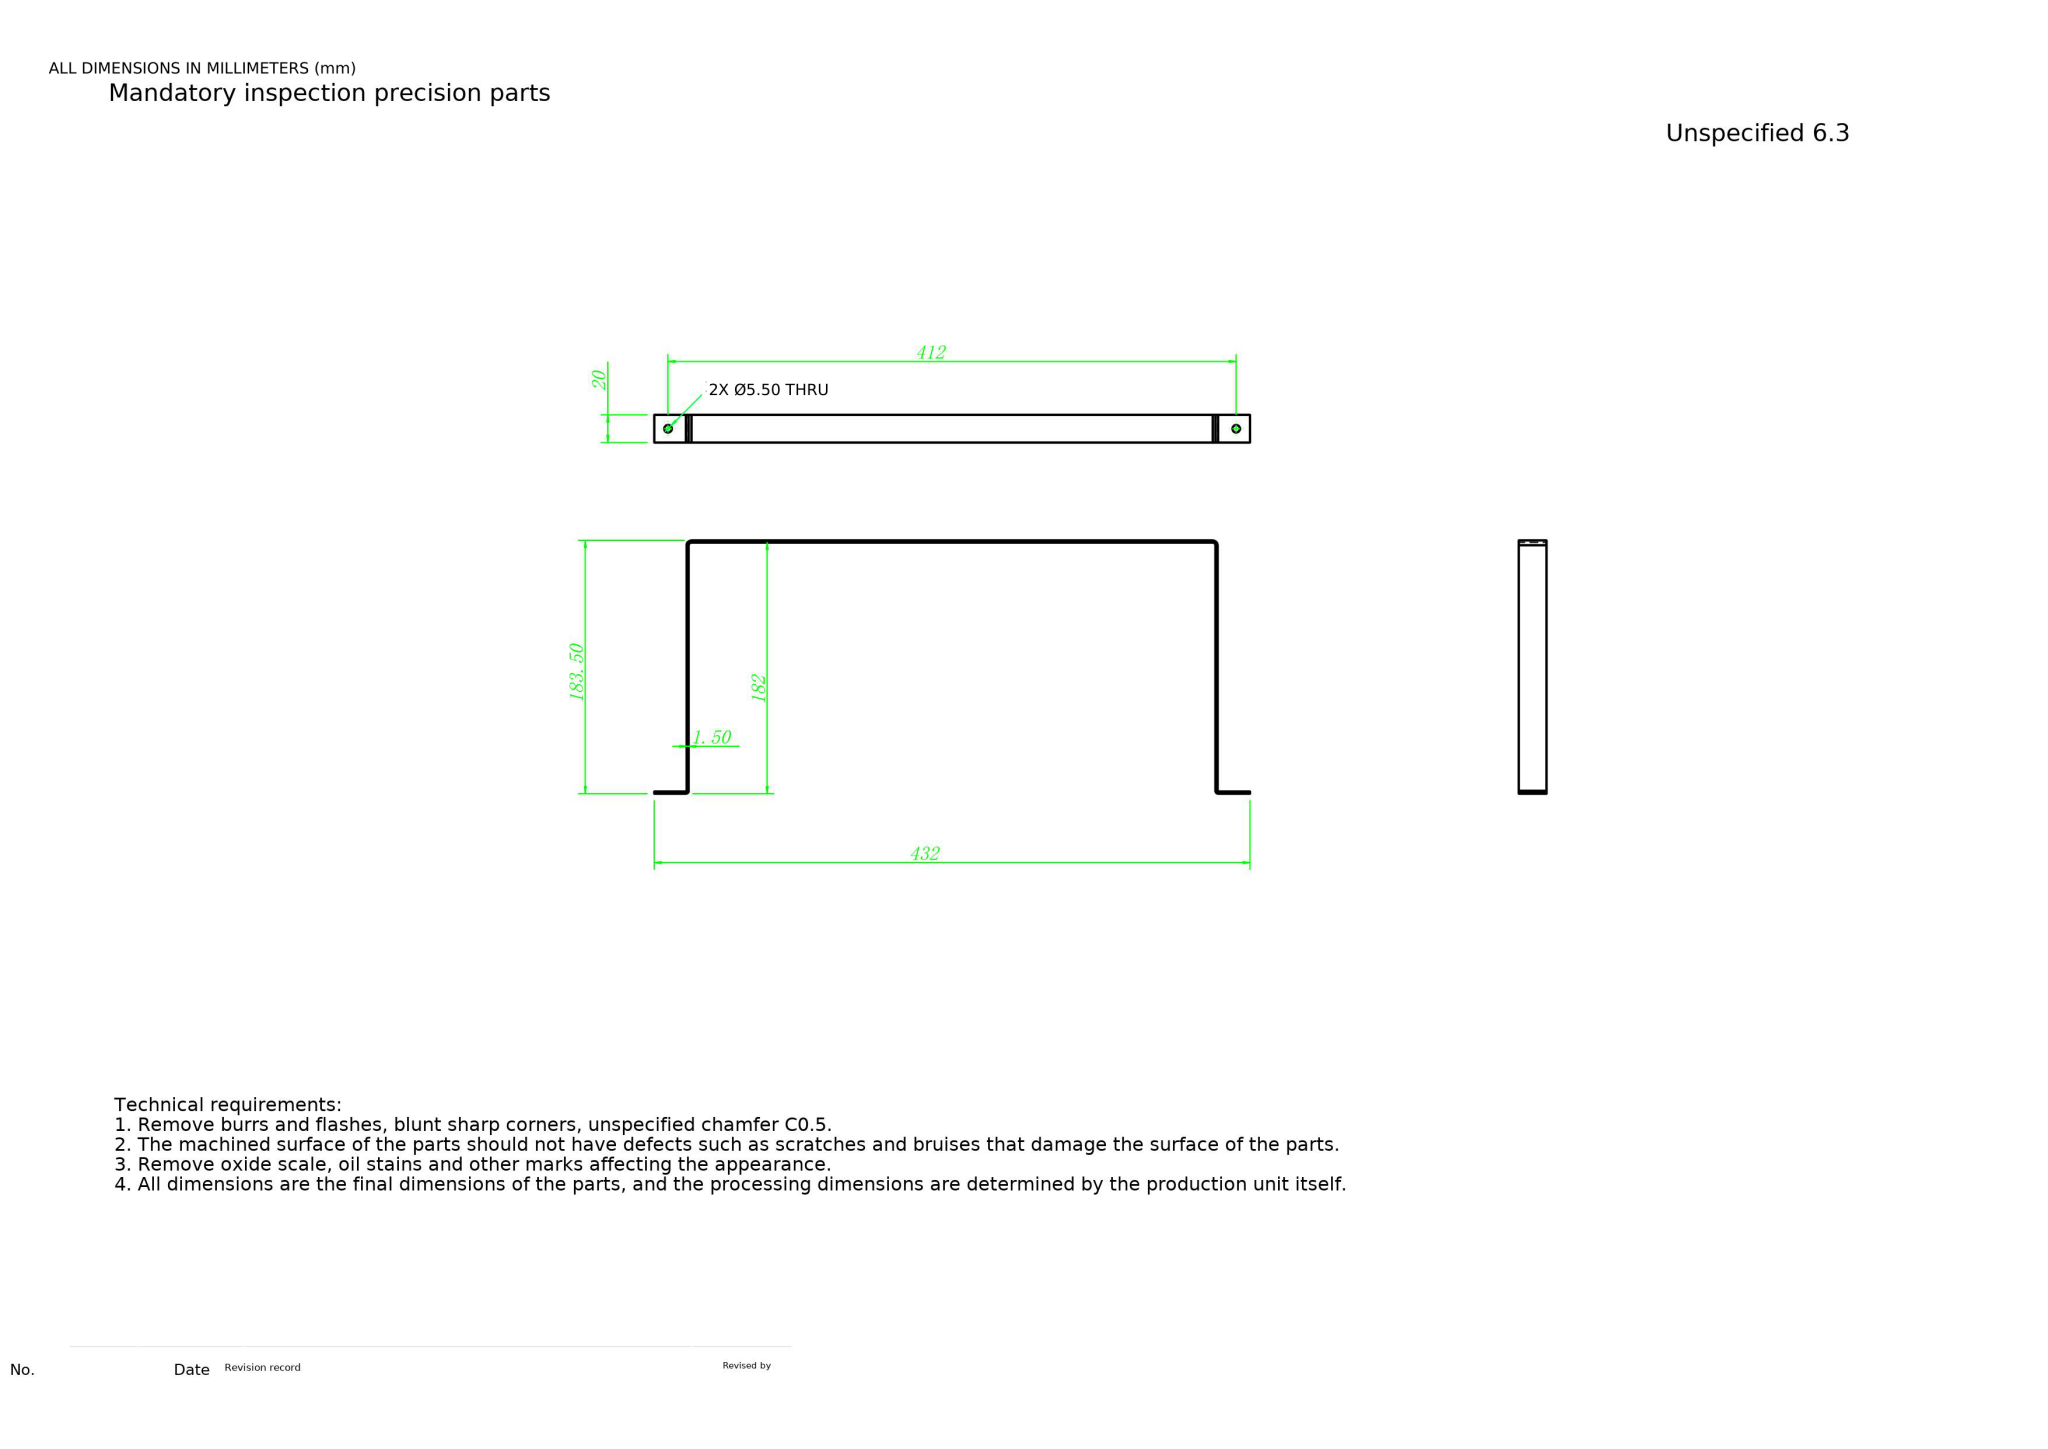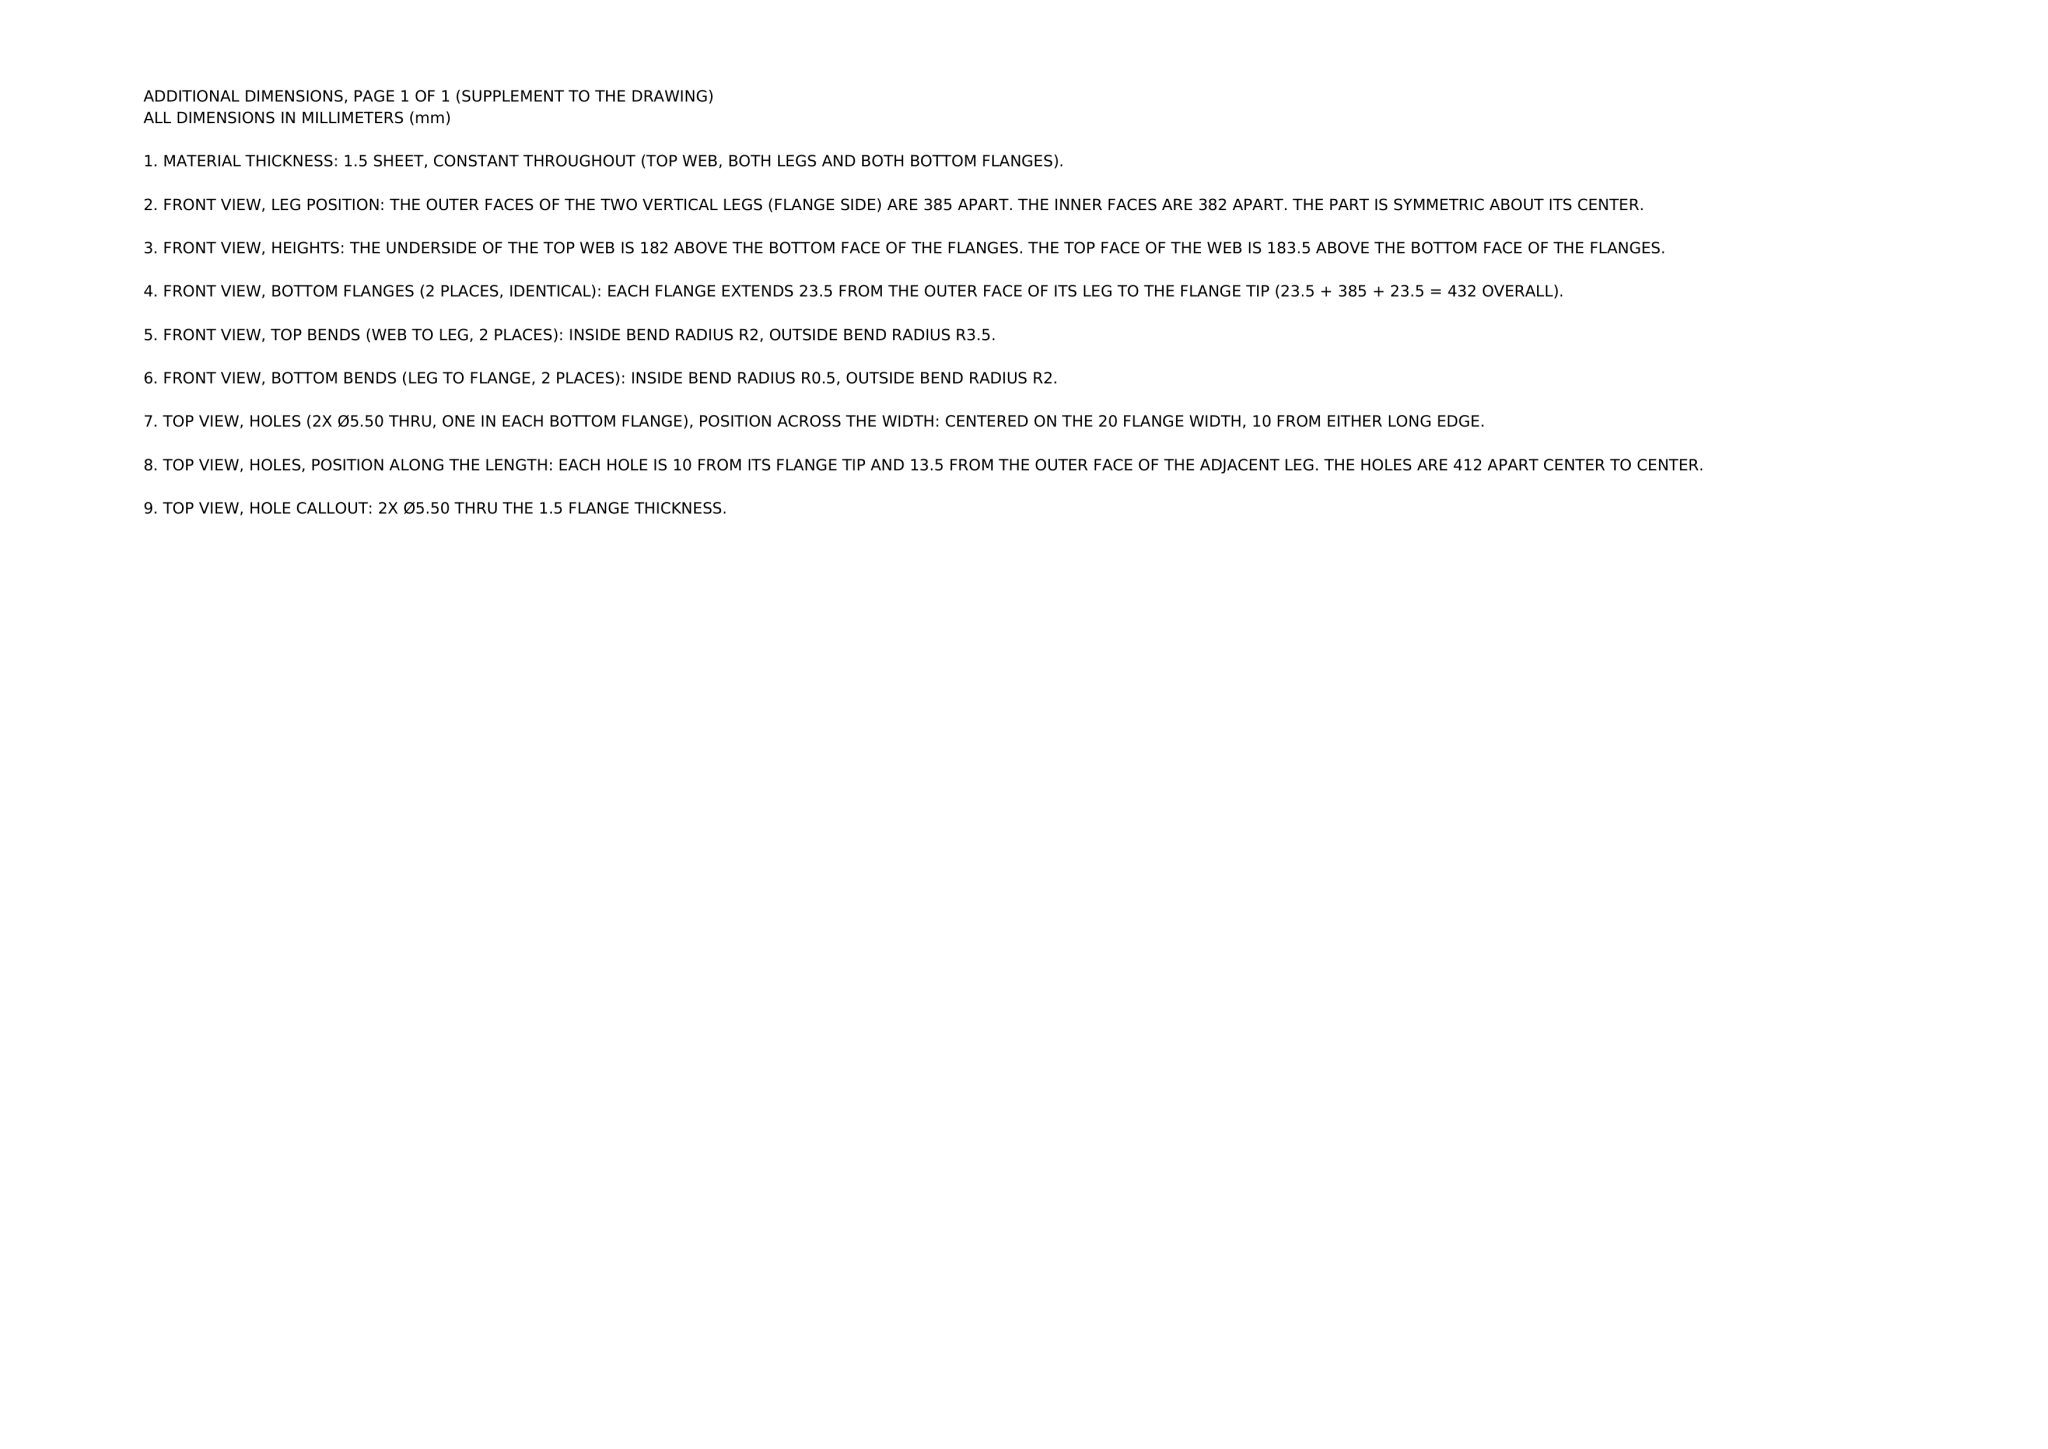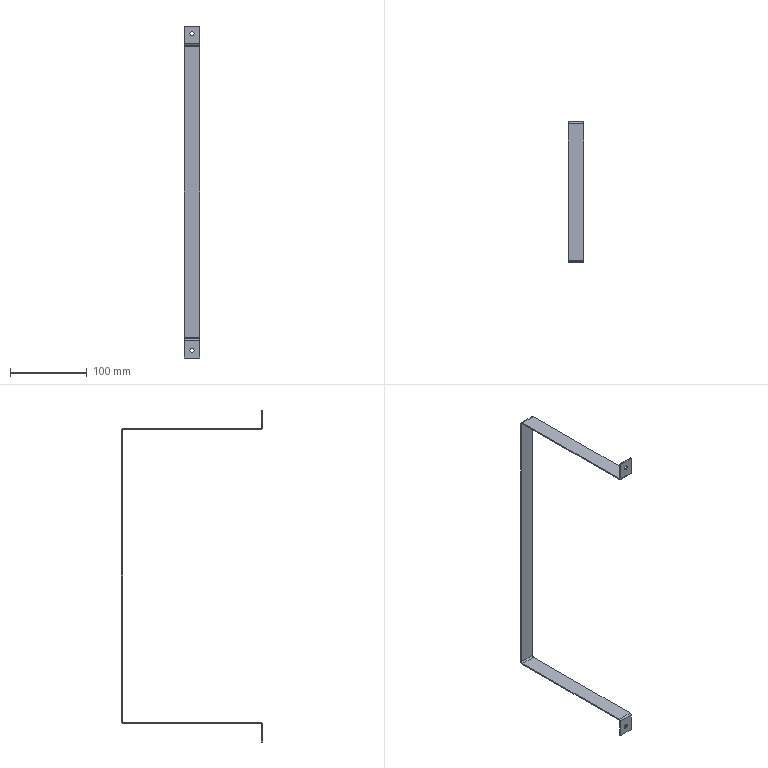Part | NX | mm | 1 solid | 26 faces | box 20 x 183.5 x 432 mm | volume 23706 mm3 | plane 14 | cylinder 12 | commonest cylinder face diameters 5.5 x4 4 x4 1 x2 7 x2
STEP:
#1=COLOUR_RGB('',0.7922,0.8196,0.9333);
#2=FILL_AREA_STYLE_COLOUR('',#1);
#3=FILL_AREA_STYLE('',(#2));
#4=SURFACE_STYLE_FILL_AREA(#3);
#5=SURFACE_SIDE_STYLE('',(#4));
#6=SURFACE_STYLE_USAGE(.BOTH.,#5);
#7=PRESENTATION_STYLE_ASSIGNMENT((#6));
#8=CARTESIAN_POINT('',(10.,0.,12.25));
#9=VERTEX_POINT('',#8);
#10=CARTESIAN_POINT('',(10.,0.,17.75));
#11=VERTEX_POINT('',#10);
#12=CARTESIAN_POINT('',(10.,0.,15.));
#13=DIRECTION('',(0.,1.,0.));
#14=DIRECTION('',(0.,0.,1.));
#15=AXIS2_PLACEMENT_3D('',#12,#13,#14);
#16=CIRCLE('',#15,2.75);
#17=EDGE_CURVE('',#9,#11,#16,.T.);
#18=ORIENTED_EDGE('',*,*,#17,.F.);
#19=CARTESIAN_POINT('',(10.,1.5,12.25));
#20=VERTEX_POINT('',#19);
#21=CARTESIAN_POINT('',(10.,1.5,12.25));
#22=DIRECTION('',(0.,1.,0.));
#23=VECTOR('',#22,1000.);
#24=LINE('',#21,#23);
#25=EDGE_CURVE('',#9,#20,#24,.T.);
#26=ORIENTED_EDGE('',*,*,#25,.T.);
#27=CARTESIAN_POINT('',(10.,1.5,17.75));
#28=VERTEX_POINT('',#27);
#29=CARTESIAN_POINT('',(10.,1.5,15.));
#30=DIRECTION('',(0.,1.,0.));
#31=DIRECTION('',(0.,0.,1.));
#32=AXIS2_PLACEMENT_3D('',#29,#30,#31);
#33=CIRCLE('',#32,2.75);
#34=EDGE_CURVE('',#20,#28,#33,.T.);
#35=ORIENTED_EDGE('',*,*,#34,.T.);
#36=CARTESIAN_POINT('',(10.,1.5,17.75));
#37=DIRECTION('',(0.,1.,0.));
#38=VECTOR('',#37,1000.);
#39=LINE('',#36,#38);
#40=EDGE_CURVE('',#11,#28,#39,.T.);
#41=ORIENTED_EDGE('',*,*,#40,.F.);
#42=EDGE_LOOP('',(#18,#26,#35,#41));
#43=FACE_OUTER_BOUND('',#42,.T.);
#44=CARTESIAN_POINT('',(10.,1.5,15.));
#45=DIRECTION('',(0.,1.,0.));
#46=DIRECTION('',(0.,0.,1.));
#47=AXIS2_PLACEMENT_3D('',#44,#45,#46);
#48=CYLINDRICAL_SURFACE('',#47,2.75);
#49=ADVANCED_FACE('',(#43),#48,.F.);
#50=CARTESIAN_POINT('',(10.,0.,-399.75));
#51=VERTEX_POINT('',#50);
#52=CARTESIAN_POINT('',(10.,0.,-394.25));
#53=VERTEX_POINT('',#52);
#54=CARTESIAN_POINT('',(10.,0.,-397.));
#55=DIRECTION('',(0.,1.,0.));
#56=DIRECTION('',(0.,0.,1.));
#57=AXIS2_PLACEMENT_3D('',#54,#55,#56);
#58=CIRCLE('',#57,2.75);
#59=EDGE_CURVE('',#51,#53,#58,.T.);
#60=ORIENTED_EDGE('',*,*,#59,.F.);
#61=CARTESIAN_POINT('',(10.,1.5,-399.75));
#62=VERTEX_POINT('',#61);
#63=CARTESIAN_POINT('',(10.,1.5,-399.75));
#64=DIRECTION('',(0.,1.,0.));
#65=VECTOR('',#64,1000.);
#66=LINE('',#63,#65);
#67=EDGE_CURVE('',#51,#62,#66,.T.);
#68=ORIENTED_EDGE('',*,*,#67,.T.);
#69=CARTESIAN_POINT('',(10.,1.5,-394.25));
#70=VERTEX_POINT('',#69);
#71=CARTESIAN_POINT('',(10.,1.5,-397.));
#72=DIRECTION('',(0.,1.,0.));
#73=DIRECTION('',(0.,0.,1.));
#74=AXIS2_PLACEMENT_3D('',#71,#72,#73);
#75=CIRCLE('',#74,2.75);
#76=EDGE_CURVE('',#62,#70,#75,.T.);
#77=ORIENTED_EDGE('',*,*,#76,.T.);
#78=CARTESIAN_POINT('',(10.,1.5,-394.25));
#79=DIRECTION('',(0.,1.,0.));
#80=VECTOR('',#79,1000.);
#81=LINE('',#78,#80);
#82=EDGE_CURVE('',#53,#70,#81,.T.);
#83=ORIENTED_EDGE('',*,*,#82,.F.);
#84=EDGE_LOOP('',(#60,#68,#77,#83));
#85=FACE_OUTER_BOUND('',#84,.T.);
#86=CARTESIAN_POINT('',(10.,1.5,-397.));
#87=DIRECTION('',(0.,1.,0.));
#88=DIRECTION('',(0.,0.,1.));
#89=AXIS2_PLACEMENT_3D('',#86,#87,#88);
#90=CYLINDRICAL_SURFACE('',#89,2.75);
#91=ADVANCED_FACE('',(#85),#90,.F.);
#92=CARTESIAN_POINT('',(10.,0.,-397.));
#93=DIRECTION('',(0.,1.,0.));
#94=DIRECTION('',(0.,0.,1.));
#95=AXIS2_PLACEMENT_3D('',#92,#93,#94);
#96=CIRCLE('',#95,2.75);
#97=EDGE_CURVE('',#53,#51,#96,.T.);
#98=ORIENTED_EDGE('',*,*,#97,.T.);
#99=ORIENTED_EDGE('',*,*,#59,.T.);
#100=EDGE_LOOP('',(#98,#99));
#101=FACE_BOUND('',#100,.T.);
#102=CARTESIAN_POINT('',(0.,-0.,-384.));
#103=VERTEX_POINT('',#102);
#104=CARTESIAN_POINT('',(0.,0.,-407.));
#105=VERTEX_POINT('',#104);
#106=CARTESIAN_POINT('',(0.,0.,-384.));
#107=DIRECTION('',(0.,0.,-1.));
#108=VECTOR('',#107,1000.);
#109=LINE('',#106,#108);
#110=EDGE_CURVE('',#103,#105,#109,.T.);
#111=ORIENTED_EDGE('',*,*,#110,.T.);
#112=CARTESIAN_POINT('',(20.,0.,-407.));
#113=VERTEX_POINT('',#112);
#114=CARTESIAN_POINT('',(20.,0.,-407.));
#115=DIRECTION('',(-1.,0.,0.));
#116=VECTOR('',#115,1000.);
#117=LINE('',#114,#116);
#118=EDGE_CURVE('',#113,#105,#117,.T.);
#119=ORIENTED_EDGE('',*,*,#118,.F.);
#120=CARTESIAN_POINT('',(20.,-0.,-384.));
#121=VERTEX_POINT('',#120);
#122=CARTESIAN_POINT('',(20.,0.,-384.));
#123=DIRECTION('',(0.,0.,-1.));
#124=VECTOR('',#123,1000.);
#125=LINE('',#122,#124);
#126=EDGE_CURVE('',#121,#113,#125,.T.);
#127=ORIENTED_EDGE('',*,*,#126,.F.);
#128=CARTESIAN_POINT('',(20.,-0.,-384.));
#129=DIRECTION('',(-1.,0.,0.));
#130=VECTOR('',#129,1000.);
#131=LINE('',#128,#130);
#132=EDGE_CURVE('',#121,#103,#131,.T.);
#133=ORIENTED_EDGE('',*,*,#132,.T.);
#134=EDGE_LOOP('',(#111,#119,#127,#133));
#135=FACE_OUTER_BOUND('',#134,.T.);
#136=CARTESIAN_POINT('',(20.,0.,-384.));
#137=DIRECTION('',(0.,1.,0.));
#138=DIRECTION('',(0.,0.,1.));
#139=AXIS2_PLACEMENT_3D('',#136,#137,#138);
#140=PLANE('',#139);
#141=ADVANCED_FACE('',(#101,#135),#140,.F.);
#142=CARTESIAN_POINT('',(0.,1.5,-407.));
#143=VERTEX_POINT('',#142);
#144=CARTESIAN_POINT('',(0.,1.5,-407.));
#145=DIRECTION('',(0.,-1.,0.));
#146=VECTOR('',#145,1000.);
#147=LINE('',#144,#146);
#148=EDGE_CURVE('',#143,#105,#147,.T.);
#149=ORIENTED_EDGE('',*,*,#148,.F.);
#150=CARTESIAN_POINT('',(20.,1.5,-407.));
#151=VERTEX_POINT('',#150);
#152=CARTESIAN_POINT('',(20.,1.5,-407.));
#153=DIRECTION('',(-1.,0.,0.));
#154=VECTOR('',#153,1000.);
#155=LINE('',#152,#154);
#156=EDGE_CURVE('',#151,#143,#155,.T.);
#157=ORIENTED_EDGE('',*,*,#156,.F.);
#158=CARTESIAN_POINT('',(20.,1.5,-407.));
#159=DIRECTION('',(0.,-1.,0.));
#160=VECTOR('',#159,1000.);
#161=LINE('',#158,#160);
#162=EDGE_CURVE('',#151,#113,#161,.T.);
#163=ORIENTED_EDGE('',*,*,#162,.T.);
#164=ORIENTED_EDGE('',*,*,#118,.T.);
#165=EDGE_LOOP('',(#149,#157,#163,#164));
#166=FACE_OUTER_BOUND('',#165,.T.);
#167=CARTESIAN_POINT('',(20.,1.5,-407.));
#168=DIRECTION('',(0.,0.,-1.));
#169=DIRECTION('',(-1.,0.,0.));
#170=AXIS2_PLACEMENT_3D('',#167,#168,#169);
#171=PLANE('',#170);
#172=ADVANCED_FACE('',(#166),#171,.T.);
#173=CARTESIAN_POINT('',(10.,1.5,-397.));
#174=DIRECTION('',(0.,1.,0.));
#175=DIRECTION('',(0.,0.,1.));
#176=AXIS2_PLACEMENT_3D('',#173,#174,#175);
#177=CIRCLE('',#176,2.75);
#178=EDGE_CURVE('',#70,#62,#177,.T.);
#179=ORIENTED_EDGE('',*,*,#178,.F.);
#180=ORIENTED_EDGE('',*,*,#76,.F.);
#181=EDGE_LOOP('',(#179,#180));
#182=FACE_BOUND('',#181,.T.);
#183=CARTESIAN_POINT('',(0.,1.5,-384.));
#184=VERTEX_POINT('',#183);
#185=CARTESIAN_POINT('',(0.,1.5,-384.));
#186=DIRECTION('',(0.,0.,-1.));
#187=VECTOR('',#186,1000.);
#188=LINE('',#185,#187);
#189=EDGE_CURVE('',#184,#143,#188,.T.);
#190=ORIENTED_EDGE('',*,*,#189,.F.);
#191=CARTESIAN_POINT('',(20.,1.5,-384.));
#192=VERTEX_POINT('',#191);
#193=CARTESIAN_POINT('',(20.,1.5,-384.));
#194=DIRECTION('',(-1.,0.,0.));
#195=VECTOR('',#194,1000.);
#196=LINE('',#193,#195);
#197=EDGE_CURVE('',#192,#184,#196,.T.);
#198=ORIENTED_EDGE('',*,*,#197,.F.);
#199=CARTESIAN_POINT('',(20.,1.5,-384.));
#200=DIRECTION('',(0.,0.,-1.));
#201=VECTOR('',#200,1000.);
#202=LINE('',#199,#201);
#203=EDGE_CURVE('',#192,#151,#202,.T.);
#204=ORIENTED_EDGE('',*,*,#203,.T.);
#205=ORIENTED_EDGE('',*,*,#156,.T.);
#206=EDGE_LOOP('',(#190,#198,#204,#205));
#207=FACE_OUTER_BOUND('',#206,.T.);
#208=CARTESIAN_POINT('',(20.,1.5,-384.));
#209=DIRECTION('',(0.,1.,0.));
#210=DIRECTION('',(0.,0.,1.));
#211=AXIS2_PLACEMENT_3D('',#208,#209,#210);
#212=PLANE('',#211);
#213=ADVANCED_FACE('',(#182,#207),#212,.T.);
#214=CARTESIAN_POINT('',(0.,2.,-383.5));
#215=VERTEX_POINT('',#214);
#216=CARTESIAN_POINT('',(0.,2.,-384.));
#217=DIRECTION('',(1.,0.,0.));
#218=DIRECTION('',(0.,0.,-1.));
#219=AXIS2_PLACEMENT_3D('',#216,#217,#218);
#220=CIRCLE('',#219,0.5);
#221=EDGE_CURVE('',#215,#184,#220,.T.);
#222=ORIENTED_EDGE('',*,*,#221,.F.);
#223=CARTESIAN_POINT('',(20.,2.,-383.5));
#224=VERTEX_POINT('',#223);
#225=CARTESIAN_POINT('',(20.,2.,-383.5));
#226=DIRECTION('',(-1.,0.,0.));
#227=VECTOR('',#226,1000.);
#228=LINE('',#225,#227);
#229=EDGE_CURVE('',#224,#215,#228,.T.);
#230=ORIENTED_EDGE('',*,*,#229,.F.);
#231=CARTESIAN_POINT('',(20.,2.,-384.));
#232=DIRECTION('',(1.,0.,0.));
#233=DIRECTION('',(0.,0.,-1.));
#234=AXIS2_PLACEMENT_3D('',#231,#232,#233);
#235=CIRCLE('',#234,0.5);
#236=EDGE_CURVE('',#224,#192,#235,.T.);
#237=ORIENTED_EDGE('',*,*,#236,.T.);
#238=ORIENTED_EDGE('',*,*,#197,.T.);
#239=EDGE_LOOP('',(#222,#230,#237,#238));
#240=FACE_OUTER_BOUND('',#239,.T.);
#241=CARTESIAN_POINT('',(20.,2.,-384.));
#242=DIRECTION('',(-1.,0.,0.));
#243=DIRECTION('',(0.,0.,1.));
#244=AXIS2_PLACEMENT_3D('',#241,#242,#243);
#245=CYLINDRICAL_SURFACE('',#244,0.5);
#246=ADVANCED_FACE('',(#240),#245,.F.);
#247=CARTESIAN_POINT('',(0.,180.,-383.5));
#248=VERTEX_POINT('',#247);
#249=CARTESIAN_POINT('',(0.,2.,-383.5));
#250=DIRECTION('',(0.,-1.,0.));
#251=VECTOR('',#250,1000.);
#252=LINE('',#249,#251);
#253=EDGE_CURVE('',#248,#215,#252,.T.);
#254=ORIENTED_EDGE('',*,*,#253,.F.);
#255=CARTESIAN_POINT('',(20.,180.,-383.5));
#256=VERTEX_POINT('',#255);
#257=CARTESIAN_POINT('',(20.,180.,-383.5));
#258=DIRECTION('',(-1.,0.,0.));
#259=VECTOR('',#258,1000.);
#260=LINE('',#257,#259);
#261=EDGE_CURVE('',#256,#248,#260,.T.);
#262=ORIENTED_EDGE('',*,*,#261,.F.);
#263=CARTESIAN_POINT('',(20.,2.,-383.5));
#264=DIRECTION('',(0.,-1.,0.));
#265=VECTOR('',#264,1000.);
#266=LINE('',#263,#265);
#267=EDGE_CURVE('',#256,#224,#266,.T.);
#268=ORIENTED_EDGE('',*,*,#267,.T.);
#269=ORIENTED_EDGE('',*,*,#229,.T.);
#270=EDGE_LOOP('',(#254,#262,#268,#269));
#271=FACE_OUTER_BOUND('',#270,.T.);
#272=CARTESIAN_POINT('',(20.,2.,-383.5));
#273=DIRECTION('',(0.,0.,-1.));
#274=DIRECTION('',(-1.,0.,0.));
#275=AXIS2_PLACEMENT_3D('',#272,#273,#274);
#276=PLANE('',#275);
#277=ADVANCED_FACE('',(#271),#276,.T.);
#278=CARTESIAN_POINT('',(0.,183.5,-380.));
#279=VERTEX_POINT('',#278);
#280=CARTESIAN_POINT('',(0.,180.,-380.));
#281=DIRECTION('',(-1.,0.,0.));
#282=DIRECTION('',(0.,0.,-1.));
#283=AXIS2_PLACEMENT_3D('',#280,#281,#282);
#284=CIRCLE('',#283,3.5);
#285=EDGE_CURVE('',#279,#248,#284,.T.);
#286=ORIENTED_EDGE('',*,*,#285,.F.);
#287=CARTESIAN_POINT('',(20.,183.5,-380.));
#288=VERTEX_POINT('',#287);
#289=CARTESIAN_POINT('',(20.,183.5,-380.));
#290=DIRECTION('',(-1.,0.,0.));
#291=VECTOR('',#290,1000.);
#292=LINE('',#289,#291);
#293=EDGE_CURVE('',#288,#279,#292,.T.);
#294=ORIENTED_EDGE('',*,*,#293,.F.);
#295=CARTESIAN_POINT('',(20.,180.,-380.));
#296=DIRECTION('',(-1.,0.,0.));
#297=DIRECTION('',(0.,0.,-1.));
#298=AXIS2_PLACEMENT_3D('',#295,#296,#297);
#299=CIRCLE('',#298,3.5);
#300=EDGE_CURVE('',#288,#256,#299,.T.);
#301=ORIENTED_EDGE('',*,*,#300,.T.);
#302=ORIENTED_EDGE('',*,*,#261,.T.);
#303=EDGE_LOOP('',(#286,#294,#301,#302));
#304=FACE_OUTER_BOUND('',#303,.T.);
#305=CARTESIAN_POINT('',(20.,180.,-380.));
#306=DIRECTION('',(-1.,0.,0.));
#307=DIRECTION('',(0.,0.,1.));
#308=AXIS2_PLACEMENT_3D('',#305,#306,#307);
#309=CYLINDRICAL_SURFACE('',#308,3.5);
#310=ADVANCED_FACE('',(#304),#309,.T.);
#311=CARTESIAN_POINT('',(0.,183.5,-2.));
#312=VERTEX_POINT('',#311);
#313=CARTESIAN_POINT('',(0.,183.5,-2.));
#314=DIRECTION('',(0.,0.,-1.));
#315=VECTOR('',#314,1000.);
#316=LINE('',#313,#315);
#317=EDGE_CURVE('',#312,#279,#316,.T.);
#318=ORIENTED_EDGE('',*,*,#317,.F.);
#319=CARTESIAN_POINT('',(20.,183.5,-2.));
#320=VERTEX_POINT('',#319);
#321=CARTESIAN_POINT('',(20.,183.5,-2.));
#322=DIRECTION('',(-1.,0.,0.));
#323=VECTOR('',#322,1000.);
#324=LINE('',#321,#323);
#325=EDGE_CURVE('',#320,#312,#324,.T.);
#326=ORIENTED_EDGE('',*,*,#325,.F.);
#327=CARTESIAN_POINT('',(20.,183.5,-2.));
#328=DIRECTION('',(0.,0.,-1.));
#329=VECTOR('',#328,1000.);
#330=LINE('',#327,#329);
#331=EDGE_CURVE('',#320,#288,#330,.T.);
#332=ORIENTED_EDGE('',*,*,#331,.T.);
#333=ORIENTED_EDGE('',*,*,#293,.T.);
#334=EDGE_LOOP('',(#318,#326,#332,#333));
#335=FACE_OUTER_BOUND('',#334,.T.);
#336=CARTESIAN_POINT('',(20.,183.5,-2.));
#337=DIRECTION('',(0.,1.,0.));
#338=DIRECTION('',(0.,0.,1.));
#339=AXIS2_PLACEMENT_3D('',#336,#337,#338);
#340=PLANE('',#339);
#341=ADVANCED_FACE('',(#335),#340,.T.);
#342=CARTESIAN_POINT('',(0.,180.,1.5));
#343=VERTEX_POINT('',#342);
#344=CARTESIAN_POINT('',(0.,180.,-2.));
#345=DIRECTION('',(-1.,0.,0.));
#346=DIRECTION('',(0.,0.,-1.));
#347=AXIS2_PLACEMENT_3D('',#344,#345,#346);
#348=CIRCLE('',#347,3.5);
#349=EDGE_CURVE('',#343,#312,#348,.T.);
#350=ORIENTED_EDGE('',*,*,#349,.F.);
#351=CARTESIAN_POINT('',(20.,180.,1.5));
#352=VERTEX_POINT('',#351);
#353=CARTESIAN_POINT('',(20.,180.,1.5));
#354=DIRECTION('',(-1.,0.,0.));
#355=VECTOR('',#354,1000.);
#356=LINE('',#353,#355);
#357=EDGE_CURVE('',#352,#343,#356,.T.);
#358=ORIENTED_EDGE('',*,*,#357,.F.);
#359=CARTESIAN_POINT('',(20.,180.,-2.));
#360=DIRECTION('',(-1.,0.,0.));
#361=DIRECTION('',(0.,0.,-1.));
#362=AXIS2_PLACEMENT_3D('',#359,#360,#361);
#363=CIRCLE('',#362,3.5);
#364=EDGE_CURVE('',#352,#320,#363,.T.);
#365=ORIENTED_EDGE('',*,*,#364,.T.);
#366=ORIENTED_EDGE('',*,*,#325,.T.);
#367=EDGE_LOOP('',(#350,#358,#365,#366));
#368=FACE_OUTER_BOUND('',#367,.T.);
#369=CARTESIAN_POINT('',(20.,180.,-2.));
#370=DIRECTION('',(-1.,0.,0.));
#371=DIRECTION('',(0.,0.,1.));
#372=AXIS2_PLACEMENT_3D('',#369,#370,#371);
#373=CYLINDRICAL_SURFACE('',#372,3.5);
#374=ADVANCED_FACE('',(#368),#373,.T.);
#375=CARTESIAN_POINT('',(0.,2.,1.5));
#376=VERTEX_POINT('',#375);
#377=CARTESIAN_POINT('',(0.,2.,1.5));
#378=DIRECTION('',(0.,1.,0.));
#379=VECTOR('',#378,1000.);
#380=LINE('',#377,#379);
#381=EDGE_CURVE('',#376,#343,#380,.T.);
#382=ORIENTED_EDGE('',*,*,#381,.F.);
#383=CARTESIAN_POINT('',(20.,2.,1.5));
#384=VERTEX_POINT('',#383);
#385=CARTESIAN_POINT('',(20.,2.,1.5));
#386=DIRECTION('',(-1.,0.,0.));
#387=VECTOR('',#386,1000.);
#388=LINE('',#385,#387);
#389=EDGE_CURVE('',#384,#376,#388,.T.);
#390=ORIENTED_EDGE('',*,*,#389,.F.);
#391=CARTESIAN_POINT('',(20.,2.,1.5));
#392=DIRECTION('',(0.,1.,0.));
#393=VECTOR('',#392,1000.);
#394=LINE('',#391,#393);
#395=EDGE_CURVE('',#384,#352,#394,.T.);
#396=ORIENTED_EDGE('',*,*,#395,.T.);
#397=ORIENTED_EDGE('',*,*,#357,.T.);
#398=EDGE_LOOP('',(#382,#390,#396,#397));
#399=FACE_OUTER_BOUND('',#398,.T.);
#400=CARTESIAN_POINT('',(20.,2.,1.5));
#401=DIRECTION('',(0.,0.,1.));
#402=DIRECTION('',(1.,0.,0.));
#403=AXIS2_PLACEMENT_3D('',#400,#401,#402);
#404=PLANE('',#403);
#405=ADVANCED_FACE('',(#399),#404,.T.);
#406=CARTESIAN_POINT('',(0.,1.5,2.));
#407=VERTEX_POINT('',#406);
#408=CARTESIAN_POINT('',(0.,2.,2.));
#409=DIRECTION('',(1.,0.,0.));
#410=DIRECTION('',(0.,0.,-1.));
#411=AXIS2_PLACEMENT_3D('',#408,#409,#410);
#412=CIRCLE('',#411,0.5);
#413=EDGE_CURVE('',#407,#376,#412,.T.);
#414=ORIENTED_EDGE('',*,*,#413,.F.);
#415=CARTESIAN_POINT('',(20.,1.5,2.));
#416=VERTEX_POINT('',#415);
#417=CARTESIAN_POINT('',(20.,1.5,2.));
#418=DIRECTION('',(-1.,0.,0.));
#419=VECTOR('',#418,1000.);
#420=LINE('',#417,#419);
#421=EDGE_CURVE('',#416,#407,#420,.T.);
#422=ORIENTED_EDGE('',*,*,#421,.F.);
#423=CARTESIAN_POINT('',(20.,2.,2.));
#424=DIRECTION('',(1.,0.,0.));
#425=DIRECTION('',(0.,0.,-1.));
#426=AXIS2_PLACEMENT_3D('',#423,#424,#425);
#427=CIRCLE('',#426,0.5);
#428=EDGE_CURVE('',#416,#384,#427,.T.);
#429=ORIENTED_EDGE('',*,*,#428,.T.);
#430=ORIENTED_EDGE('',*,*,#389,.T.);
#431=EDGE_LOOP('',(#414,#422,#429,#430));
#432=FACE_OUTER_BOUND('',#431,.T.);
#433=CARTESIAN_POINT('',(20.,2.,2.));
#434=DIRECTION('',(-1.,0.,0.));
#435=DIRECTION('',(0.,0.,1.));
#436=AXIS2_PLACEMENT_3D('',#433,#434,#435);
#437=CYLINDRICAL_SURFACE('',#436,0.5);
#438=ADVANCED_FACE('',(#432),#437,.F.);
#439=CARTESIAN_POINT('',(10.,1.5,15.));
#440=DIRECTION('',(0.,1.,0.));
#441=DIRECTION('',(0.,0.,1.));
#442=AXIS2_PLACEMENT_3D('',#439,#440,#441);
#443=CIRCLE('',#442,2.75);
#444=EDGE_CURVE('',#28,#20,#443,.T.);
#445=ORIENTED_EDGE('',*,*,#444,.F.);
#446=ORIENTED_EDGE('',*,*,#34,.F.);
#447=EDGE_LOOP('',(#445,#446));
#448=FACE_BOUND('',#447,.T.);
#449=CARTESIAN_POINT('',(0.,1.5,25.));
#450=VERTEX_POINT('',#449);
#451=CARTESIAN_POINT('',(0.,1.5,2.));
#452=DIRECTION('',(0.,0.,-1.));
#453=VECTOR('',#452,1000.);
#454=LINE('',#451,#453);
#455=EDGE_CURVE('',#450,#407,#454,.T.);
#456=ORIENTED_EDGE('',*,*,#455,.F.);
#457=CARTESIAN_POINT('',(20.,1.5,25.));
#458=VERTEX_POINT('',#457);
#459=CARTESIAN_POINT('',(20.,1.5,25.));
#460=DIRECTION('',(-1.,0.,0.));
#461=VECTOR('',#460,1000.);
#462=LINE('',#459,#461);
#463=EDGE_CURVE('',#458,#450,#462,.T.);
#464=ORIENTED_EDGE('',*,*,#463,.F.);
#465=CARTESIAN_POINT('',(20.,1.5,2.));
#466=DIRECTION('',(0.,0.,-1.));
#467=VECTOR('',#466,1000.);
#468=LINE('',#465,#467);
#469=EDGE_CURVE('',#458,#416,#468,.T.);
#470=ORIENTED_EDGE('',*,*,#469,.T.);
#471=ORIENTED_EDGE('',*,*,#421,.T.);
#472=EDGE_LOOP('',(#456,#464,#470,#471));
#473=FACE_OUTER_BOUND('',#472,.T.);
#474=CARTESIAN_POINT('',(20.,1.5,2.));
#475=DIRECTION('',(0.,1.,0.));
#476=DIRECTION('',(0.,0.,1.));
#477=AXIS2_PLACEMENT_3D('',#474,#475,#476);
#478=PLANE('',#477);
#479=ADVANCED_FACE('',(#448,#473),#478,.T.);
#480=CARTESIAN_POINT('',(0.,0.,25.));
#481=VERTEX_POINT('',#480);
#482=CARTESIAN_POINT('',(0.,0.,25.));
#483=DIRECTION('',(0.,1.,0.));
#484=VECTOR('',#483,1000.);
#485=LINE('',#482,#484);
#486=EDGE_CURVE('',#481,#450,#485,.T.);
#487=ORIENTED_EDGE('',*,*,#486,.F.);
#488=CARTESIAN_POINT('',(20.,0.,25.));
#489=VERTEX_POINT('',#488);
#490=CARTESIAN_POINT('',(20.,0.,25.));
#491=DIRECTION('',(-1.,0.,0.));
#492=VECTOR('',#491,1000.);
#493=LINE('',#490,#492);
#494=EDGE_CURVE('',#489,#481,#493,.T.);
#495=ORIENTED_EDGE('',*,*,#494,.F.);
#496=CARTESIAN_POINT('',(20.,0.,25.));
#497=DIRECTION('',(0.,1.,0.));
#498=VECTOR('',#497,1000.);
#499=LINE('',#496,#498);
#500=EDGE_CURVE('',#489,#458,#499,.T.);
#501=ORIENTED_EDGE('',*,*,#500,.T.);
#502=ORIENTED_EDGE('',*,*,#463,.T.);
#503=EDGE_LOOP('',(#487,#495,#501,#502));
#504=FACE_OUTER_BOUND('',#503,.T.);
#505=CARTESIAN_POINT('',(20.,0.,25.));
#506=DIRECTION('',(0.,0.,1.));
#507=DIRECTION('',(1.,0.,0.));
#508=AXIS2_PLACEMENT_3D('',#505,#506,#507);
#509=PLANE('',#508);
#510=ADVANCED_FACE('',(#504),#509,.T.);
#511=CARTESIAN_POINT('',(10.,0.,15.));
#512=DIRECTION('',(0.,1.,0.));
#513=DIRECTION('',(0.,0.,1.));
#514=AXIS2_PLACEMENT_3D('',#511,#512,#513);
#515=CIRCLE('',#514,2.75);
#516=EDGE_CURVE('',#11,#9,#515,.T.);
#517=ORIENTED_EDGE('',*,*,#516,.T.);
#518=ORIENTED_EDGE('',*,*,#17,.T.);
#519=EDGE_LOOP('',(#517,#518));
#520=FACE_BOUND('',#519,.T.);
#521=CARTESIAN_POINT('',(0.,0.,2.));
#522=VERTEX_POINT('',#521);
#523=CARTESIAN_POINT('',(0.,0.,2.));
#524=DIRECTION('',(0.,0.,-1.));
#525=VECTOR('',#524,1000.);
#526=LINE('',#523,#525);
#527=EDGE_CURVE('',#481,#522,#526,.T.);
#528=ORIENTED_EDGE('',*,*,#527,.T.);
#529=CARTESIAN_POINT('',(20.,0.,2.));
#530=VERTEX_POINT('',#529);
#531=CARTESIAN_POINT('',(20.,0.,2.));
#532=DIRECTION('',(-1.,0.,0.));
#533=VECTOR('',#532,1000.);
#534=LINE('',#531,#533);
#535=EDGE_CURVE('',#530,#522,#534,.T.);
#536=ORIENTED_EDGE('',*,*,#535,.F.);
#537=CARTESIAN_POINT('',(20.,0.,2.));
#538=DIRECTION('',(0.,0.,-1.));
#539=VECTOR('',#538,1000.);
#540=LINE('',#537,#539);
#541=EDGE_CURVE('',#489,#530,#540,.T.);
#542=ORIENTED_EDGE('',*,*,#541,.F.);
#543=ORIENTED_EDGE('',*,*,#494,.T.);
#544=EDGE_LOOP('',(#528,#536,#542,#543));
#545=FACE_OUTER_BOUND('',#544,.T.);
#546=CARTESIAN_POINT('',(20.,0.,2.));
#547=DIRECTION('',(0.,1.,0.));
#548=DIRECTION('',(0.,0.,1.));
#549=AXIS2_PLACEMENT_3D('',#546,#547,#548);
#550=PLANE('',#549);
#551=ADVANCED_FACE('',(#520,#545),#550,.F.);
#552=CARTESIAN_POINT('',(0.,2.,0.));
#553=VERTEX_POINT('',#552);
#554=CARTESIAN_POINT('',(0.,2.,2.));
#555=DIRECTION('',(1.,0.,0.));
#556=DIRECTION('',(0.,0.,-1.));
#557=AXIS2_PLACEMENT_3D('',#554,#555,#556);
#558=CIRCLE('',#557,2.);
#559=EDGE_CURVE('',#522,#553,#558,.T.);
#560=ORIENTED_EDGE('',*,*,#559,.T.);
#561=CARTESIAN_POINT('',(20.,2.,0.));
#562=VERTEX_POINT('',#561);
#563=CARTESIAN_POINT('',(20.,2.,0.));
#564=DIRECTION('',(-1.,0.,0.));
#565=VECTOR('',#564,1000.);
#566=LINE('',#563,#565);
#567=EDGE_CURVE('',#562,#553,#566,.T.);
#568=ORIENTED_EDGE('',*,*,#567,.F.);
#569=CARTESIAN_POINT('',(20.,2.,2.));
#570=DIRECTION('',(1.,0.,0.));
#571=DIRECTION('',(0.,0.,-1.));
#572=AXIS2_PLACEMENT_3D('',#569,#570,#571);
#573=CIRCLE('',#572,2.);
#574=EDGE_CURVE('',#530,#562,#573,.T.);
#575=ORIENTED_EDGE('',*,*,#574,.F.);
#576=ORIENTED_EDGE('',*,*,#535,.T.);
#577=EDGE_LOOP('',(#560,#568,#575,#576));
#578=FACE_OUTER_BOUND('',#577,.T.);
#579=CARTESIAN_POINT('',(20.,2.,2.));
#580=DIRECTION('',(-1.,0.,0.));
#581=DIRECTION('',(0.,0.,1.));
#582=AXIS2_PLACEMENT_3D('',#579,#580,#581);
#583=CYLINDRICAL_SURFACE('',#582,2.);
#584=ADVANCED_FACE('',(#578),#583,.T.);
#585=CARTESIAN_POINT('',(0.,180.,0.));
#586=VERTEX_POINT('',#585);
#587=CARTESIAN_POINT('',(0.,2.,0.));
#588=DIRECTION('',(0.,1.,0.));
#589=VECTOR('',#588,1000.);
#590=LINE('',#587,#589);
#591=EDGE_CURVE('',#553,#586,#590,.T.);
#592=ORIENTED_EDGE('',*,*,#591,.T.);
#593=CARTESIAN_POINT('',(20.,180.,0.));
#594=VERTEX_POINT('',#593);
#595=CARTESIAN_POINT('',(20.,180.,0.));
#596=DIRECTION('',(-1.,0.,0.));
#597=VECTOR('',#596,1000.);
#598=LINE('',#595,#597);
#599=EDGE_CURVE('',#594,#586,#598,.T.);
#600=ORIENTED_EDGE('',*,*,#599,.F.);
#601=CARTESIAN_POINT('',(20.,2.,0.));
#602=DIRECTION('',(0.,1.,0.));
#603=VECTOR('',#602,1000.);
#604=LINE('',#601,#603);
#605=EDGE_CURVE('',#562,#594,#604,.T.);
#606=ORIENTED_EDGE('',*,*,#605,.F.);
#607=ORIENTED_EDGE('',*,*,#567,.T.);
#608=EDGE_LOOP('',(#592,#600,#606,#607));
#609=FACE_OUTER_BOUND('',#608,.T.);
#610=CARTESIAN_POINT('',(20.,2.,0.));
#611=DIRECTION('',(0.,0.,1.));
#612=DIRECTION('',(1.,0.,0.));
#613=AXIS2_PLACEMENT_3D('',#610,#611,#612);
#614=PLANE('',#613);
#615=ADVANCED_FACE('',(#609),#614,.F.);
#616=CARTESIAN_POINT('',(0.,182.,-2.));
#617=VERTEX_POINT('',#616);
#618=CARTESIAN_POINT('',(0.,180.,-2.));
#619=DIRECTION('',(-1.,0.,0.));
#620=DIRECTION('',(0.,0.,1.));
#621=AXIS2_PLACEMENT_3D('',#618,#619,#620);
#622=CIRCLE('',#621,2.);
#623=EDGE_CURVE('',#586,#617,#622,.T.);
#624=ORIENTED_EDGE('',*,*,#623,.T.);
#625=CARTESIAN_POINT('',(20.,182.,-2.));
#626=VERTEX_POINT('',#625);
#627=CARTESIAN_POINT('',(20.,182.,-2.));
#628=DIRECTION('',(-1.,0.,0.));
#629=VECTOR('',#628,1000.);
#630=LINE('',#627,#629);
#631=EDGE_CURVE('',#626,#617,#630,.T.);
#632=ORIENTED_EDGE('',*,*,#631,.F.);
#633=CARTESIAN_POINT('',(20.,180.,-2.));
#634=DIRECTION('',(-1.,0.,0.));
#635=DIRECTION('',(0.,0.,1.));
#636=AXIS2_PLACEMENT_3D('',#633,#634,#635);
#637=CIRCLE('',#636,2.);
#638=EDGE_CURVE('',#594,#626,#637,.T.);
#639=ORIENTED_EDGE('',*,*,#638,.F.);
#640=ORIENTED_EDGE('',*,*,#599,.T.);
#641=EDGE_LOOP('',(#624,#632,#639,#640));
#642=FACE_OUTER_BOUND('',#641,.T.);
#643=CARTESIAN_POINT('',(20.,180.,-2.));
#644=DIRECTION('',(-1.,0.,0.));
#645=DIRECTION('',(0.,0.,1.));
#646=AXIS2_PLACEMENT_3D('',#643,#644,#645);
#647=CYLINDRICAL_SURFACE('',#646,2.);
#648=ADVANCED_FACE('',(#642),#647,.F.);
#649=CARTESIAN_POINT('',(0.,182.,-380.));
#650=VERTEX_POINT('',#649);
#651=CARTESIAN_POINT('',(0.,182.,-2.));
#652=DIRECTION('',(0.,0.,-1.));
#653=VECTOR('',#652,1000.);
#654=LINE('',#651,#653);
#655=EDGE_CURVE('',#617,#650,#654,.T.);
#656=ORIENTED_EDGE('',*,*,#655,.T.);
#657=CARTESIAN_POINT('',(20.,182.,-380.));
#658=VERTEX_POINT('',#657);
#659=CARTESIAN_POINT('',(20.,182.,-380.));
#660=DIRECTION('',(-1.,0.,0.));
#661=VECTOR('',#660,1000.);
#662=LINE('',#659,#661);
#663=EDGE_CURVE('',#658,#650,#662,.T.);
#664=ORIENTED_EDGE('',*,*,#663,.F.);
#665=CARTESIAN_POINT('',(20.,182.,-2.));
#666=DIRECTION('',(0.,0.,-1.));
#667=VECTOR('',#666,1000.);
#668=LINE('',#665,#667);
#669=EDGE_CURVE('',#626,#658,#668,.T.);
#670=ORIENTED_EDGE('',*,*,#669,.F.);
#671=ORIENTED_EDGE('',*,*,#631,.T.);
#672=EDGE_LOOP('',(#656,#664,#670,#671));
#673=FACE_OUTER_BOUND('',#672,.T.);
#674=CARTESIAN_POINT('',(20.,182.,-2.));
#675=DIRECTION('',(0.,1.,0.));
#676=DIRECTION('',(0.,0.,1.));
#677=AXIS2_PLACEMENT_3D('',#674,#675,#676);
#678=PLANE('',#677);
#679=ADVANCED_FACE('',(#673),#678,.F.);
#680=CARTESIAN_POINT('',(0.,180.,-382.));
#681=VERTEX_POINT('',#680);
#682=CARTESIAN_POINT('',(0.,180.,-380.));
#683=DIRECTION('',(-1.,0.,0.));
#684=DIRECTION('',(0.,0.,1.));
#685=AXIS2_PLACEMENT_3D('',#682,#683,#684);
#686=CIRCLE('',#685,2.);
#687=EDGE_CURVE('',#650,#681,#686,.T.);
#688=ORIENTED_EDGE('',*,*,#687,.T.);
#689=CARTESIAN_POINT('',(20.,180.,-382.));
#690=VERTEX_POINT('',#689);
#691=CARTESIAN_POINT('',(20.,180.,-382.));
#692=DIRECTION('',(-1.,0.,0.));
#693=VECTOR('',#692,1000.);
#694=LINE('',#691,#693);
#695=EDGE_CURVE('',#690,#681,#694,.T.);
#696=ORIENTED_EDGE('',*,*,#695,.F.);
#697=CARTESIAN_POINT('',(20.,180.,-380.));
#698=DIRECTION('',(-1.,0.,0.));
#699=DIRECTION('',(0.,0.,1.));
#700=AXIS2_PLACEMENT_3D('',#697,#698,#699);
#701=CIRCLE('',#700,2.);
#702=EDGE_CURVE('',#658,#690,#701,.T.);
#703=ORIENTED_EDGE('',*,*,#702,.F.);
#704=ORIENTED_EDGE('',*,*,#663,.T.);
#705=EDGE_LOOP('',(#688,#696,#703,#704));
#706=FACE_OUTER_BOUND('',#705,.T.);
#707=CARTESIAN_POINT('',(20.,180.,-380.));
#708=DIRECTION('',(-1.,0.,0.));
#709=DIRECTION('',(0.,0.,1.));
#710=AXIS2_PLACEMENT_3D('',#707,#708,#709);
#711=CYLINDRICAL_SURFACE('',#710,2.);
#712=ADVANCED_FACE('',(#706),#711,.F.);
#713=CARTESIAN_POINT('',(0.,2.,-382.));
#714=VERTEX_POINT('',#713);
#715=CARTESIAN_POINT('',(0.,2.,-382.));
#716=DIRECTION('',(0.,-1.,0.));
#717=VECTOR('',#716,1000.);
#718=LINE('',#715,#717);
#719=EDGE_CURVE('',#681,#714,#718,.T.);
#720=ORIENTED_EDGE('',*,*,#719,.T.);
#721=CARTESIAN_POINT('',(20.,2.,-382.));
#722=VERTEX_POINT('',#721);
#723=CARTESIAN_POINT('',(20.,2.,-382.));
#724=DIRECTION('',(-1.,0.,0.));
#725=VECTOR('',#724,1000.);
#726=LINE('',#723,#725);
#727=EDGE_CURVE('',#722,#714,#726,.T.);
#728=ORIENTED_EDGE('',*,*,#727,.F.);
#729=CARTESIAN_POINT('',(20.,2.,-382.));
#730=DIRECTION('',(0.,-1.,0.));
#731=VECTOR('',#730,1000.);
#732=LINE('',#729,#731);
#733=EDGE_CURVE('',#690,#722,#732,.T.);
#734=ORIENTED_EDGE('',*,*,#733,.F.);
#735=ORIENTED_EDGE('',*,*,#695,.T.);
#736=EDGE_LOOP('',(#720,#728,#734,#735));
#737=FACE_OUTER_BOUND('',#736,.T.);
#738=CARTESIAN_POINT('',(20.,2.,-382.));
#739=DIRECTION('',(0.,0.,-1.));
#740=DIRECTION('',(-1.,0.,0.));
#741=AXIS2_PLACEMENT_3D('',#738,#739,#740);
#742=PLANE('',#741);
#743=ADVANCED_FACE('',(#737),#742,.F.);
#744=CARTESIAN_POINT('',(0.,2.,-384.));
#745=DIRECTION('',(1.,0.,0.));
#746=DIRECTION('',(0.,0.,1.));
#747=AXIS2_PLACEMENT_3D('',#744,#745,#746);
#748=CIRCLE('',#747,2.);
#749=EDGE_CURVE('',#714,#103,#748,.T.);
#750=ORIENTED_EDGE('',*,*,#749,.T.);
#751=ORIENTED_EDGE('',*,*,#132,.F.);
#752=CARTESIAN_POINT('',(20.,2.,-384.));
#753=DIRECTION('',(1.,0.,0.));
#754=DIRECTION('',(0.,0.,1.));
#755=AXIS2_PLACEMENT_3D('',#752,#753,#754);
#756=CIRCLE('',#755,2.);
#757=EDGE_CURVE('',#722,#121,#756,.T.);
#758=ORIENTED_EDGE('',*,*,#757,.F.);
#759=ORIENTED_EDGE('',*,*,#727,.T.);
#760=EDGE_LOOP('',(#750,#751,#758,#759));
#761=FACE_OUTER_BOUND('',#760,.T.);
#762=CARTESIAN_POINT('',(20.,2.,-384.));
#763=DIRECTION('',(-1.,0.,0.));
#764=DIRECTION('',(0.,0.,1.));
#765=AXIS2_PLACEMENT_3D('',#762,#763,#764);
#766=CYLINDRICAL_SURFACE('',#765,2.);
#767=ADVANCED_FACE('',(#761),#766,.T.);
#768=ORIENTED_EDGE('',*,*,#126,.T.);
#769=ORIENTED_EDGE('',*,*,#162,.F.);
#770=ORIENTED_EDGE('',*,*,#203,.F.);
#771=ORIENTED_EDGE('',*,*,#236,.F.);
#772=ORIENTED_EDGE('',*,*,#267,.F.);
#773=ORIENTED_EDGE('',*,*,#300,.F.);
#774=ORIENTED_EDGE('',*,*,#331,.F.);
#775=ORIENTED_EDGE('',*,*,#364,.F.);
#776=ORIENTED_EDGE('',*,*,#395,.F.);
#777=ORIENTED_EDGE('',*,*,#428,.F.);
#778=ORIENTED_EDGE('',*,*,#469,.F.);
#779=ORIENTED_EDGE('',*,*,#500,.F.);
#780=ORIENTED_EDGE('',*,*,#541,.T.);
#781=ORIENTED_EDGE('',*,*,#574,.T.);
#782=ORIENTED_EDGE('',*,*,#605,.T.);
#783=ORIENTED_EDGE('',*,*,#638,.T.);
#784=ORIENTED_EDGE('',*,*,#669,.T.);
#785=ORIENTED_EDGE('',*,*,#702,.T.);
#786=ORIENTED_EDGE('',*,*,#733,.T.);
#787=ORIENTED_EDGE('',*,*,#757,.T.);
#788=EDGE_LOOP('',(#768,#769,#770,#771,#772,#773,#774,#775,#776,#777,#778,#779,#780,#781,#782,#783,#784,#785,#786,#787));
#789=FACE_OUTER_BOUND('',#788,.T.);
#790=CARTESIAN_POINT('',(20.,2.,-384.));
#791=DIRECTION('',(1.,0.,0.));
#792=DIRECTION('',(0.,0.,-1.));
#793=AXIS2_PLACEMENT_3D('',#790,#791,#792);
#794=PLANE('',#793);
#795=ADVANCED_FACE('',(#789),#794,.T.);
#796=ORIENTED_EDGE('',*,*,#110,.F.);
#797=ORIENTED_EDGE('',*,*,#749,.F.);
#798=ORIENTED_EDGE('',*,*,#719,.F.);
#799=ORIENTED_EDGE('',*,*,#687,.F.);
#800=ORIENTED_EDGE('',*,*,#655,.F.);
#801=ORIENTED_EDGE('',*,*,#623,.F.);
#802=ORIENTED_EDGE('',*,*,#591,.F.);
#803=ORIENTED_EDGE('',*,*,#559,.F.);
#804=ORIENTED_EDGE('',*,*,#527,.F.);
#805=ORIENTED_EDGE('',*,*,#486,.T.);
#806=ORIENTED_EDGE('',*,*,#455,.T.);
#807=ORIENTED_EDGE('',*,*,#413,.T.);
#808=ORIENTED_EDGE('',*,*,#381,.T.);
#809=ORIENTED_EDGE('',*,*,#349,.T.);
#810=ORIENTED_EDGE('',*,*,#317,.T.);
#811=ORIENTED_EDGE('',*,*,#285,.T.);
#812=ORIENTED_EDGE('',*,*,#253,.T.);
#813=ORIENTED_EDGE('',*,*,#221,.T.);
#814=ORIENTED_EDGE('',*,*,#189,.T.);
#815=ORIENTED_EDGE('',*,*,#148,.T.);
#816=EDGE_LOOP('',(#796,#797,#798,#799,#800,#801,#802,#803,#804,#805,#806,#807,#808,#809,#810,#811,#812,#813,#814,#815));
#817=FACE_OUTER_BOUND('',#816,.T.);
#818=CARTESIAN_POINT('',(0.,2.,-384.));
#819=DIRECTION('',(1.,0.,0.));
#820=DIRECTION('',(0.,0.,-1.));
#821=AXIS2_PLACEMENT_3D('',#818,#819,#820);
#822=PLANE('',#821);
#823=ADVANCED_FACE('',(#817),#822,.F.);
#824=ORIENTED_EDGE('',*,*,#67,.F.);
#825=ORIENTED_EDGE('',*,*,#97,.F.);
#826=ORIENTED_EDGE('',*,*,#82,.T.);
#827=ORIENTED_EDGE('',*,*,#178,.T.);
#828=EDGE_LOOP('',(#824,#825,#826,#827));
#829=FACE_OUTER_BOUND('',#828,.T.);
#830=CARTESIAN_POINT('',(10.,1.5,-397.));
#831=DIRECTION('',(0.,1.,0.));
#832=DIRECTION('',(0.,0.,1.));
#833=AXIS2_PLACEMENT_3D('',#830,#831,#832);
#834=CYLINDRICAL_SURFACE('',#833,2.75);
#835=ADVANCED_FACE('',(#829),#834,.F.);
#836=ORIENTED_EDGE('',*,*,#25,.F.);
#837=ORIENTED_EDGE('',*,*,#516,.F.);
#838=ORIENTED_EDGE('',*,*,#40,.T.);
#839=ORIENTED_EDGE('',*,*,#444,.T.);
#840=EDGE_LOOP('',(#836,#837,#838,#839));
#841=FACE_OUTER_BOUND('',#840,.T.);
#842=CARTESIAN_POINT('',(10.,1.5,15.));
#843=DIRECTION('',(0.,1.,0.));
#844=DIRECTION('',(0.,0.,1.));
#845=AXIS2_PLACEMENT_3D('',#842,#843,#844);
#846=CYLINDRICAL_SURFACE('',#845,2.75);
#847=ADVANCED_FACE('',(#841),#846,.F.);
#848=CLOSED_SHELL('',(#49,#91,#141,#172,#213,#246,#277,#310,#341,#374,#405,#438,#479,#510,#551,#584,#615,#648,#679,#712,#743,#767,#795,#823,#835,#847));
#849=MANIFOLD_SOLID_BREP('',#848);
#850=STYLED_ITEM('',(#7),#849);
#851=PRESENTATION_LAYER_ASSIGNMENT('','',(#850));
#852=CARTESIAN_POINT('',(0.,0.,0.));
#853=DIRECTION('',(0.,0.,1.));
#854=DIRECTION('',(1.,0.,0.));
#855=AXIS2_PLACEMENT_3D('',#852,#853,#854);
#856=(LENGTH_UNIT()NAMED_UNIT(*)SI_UNIT(.MILLI.,.METRE.));
#857=UNCERTAINTY_MEASURE_WITH_UNIT(LENGTH_MEASURE(0.00001),#856,'','');
#858=(NAMED_UNIT(*)PLANE_ANGLE_UNIT()SI_UNIT($,.RADIAN.));
#859=(NAMED_UNIT(*)SI_UNIT($,.STERADIAN.)SOLID_ANGLE_UNIT());
#860=(GEOMETRIC_REPRESENTATION_CONTEXT(3)GLOBAL_UNCERTAINTY_ASSIGNED_CONTEXT((#857))GLOBAL_UNIT_ASSIGNED_CONTEXT((#856,#858,#859))REPRESENTATION_CONTEXT('',''));
#861=ADVANCED_BREP_SHAPE_REPRESENTATION('',(#849,#855),#860);
#862=(LENGTH_UNIT()NAMED_UNIT(*)SI_UNIT(.MILLI.,.METRE.));
#863=UNCERTAINTY_MEASURE_WITH_UNIT(LENGTH_MEASURE(0.00001),#862,'','');
#864=(NAMED_UNIT(*)PLANE_ANGLE_UNIT()SI_UNIT($,.RADIAN.));
#865=(NAMED_UNIT(*)SI_UNIT($,.STERADIAN.)SOLID_ANGLE_UNIT());
#866=(GEOMETRIC_REPRESENTATION_CONTEXT(3)GLOBAL_UNCERTAINTY_ASSIGNED_CONTEXT((#863))GLOBAL_UNIT_ASSIGNED_CONTEXT((#862,#864,#865))REPRESENTATION_CONTEXT('',''));
#867=MECHANICAL_DESIGN_GEOMETRIC_PRESENTATION_REPRESENTATION('',(#850),#866);